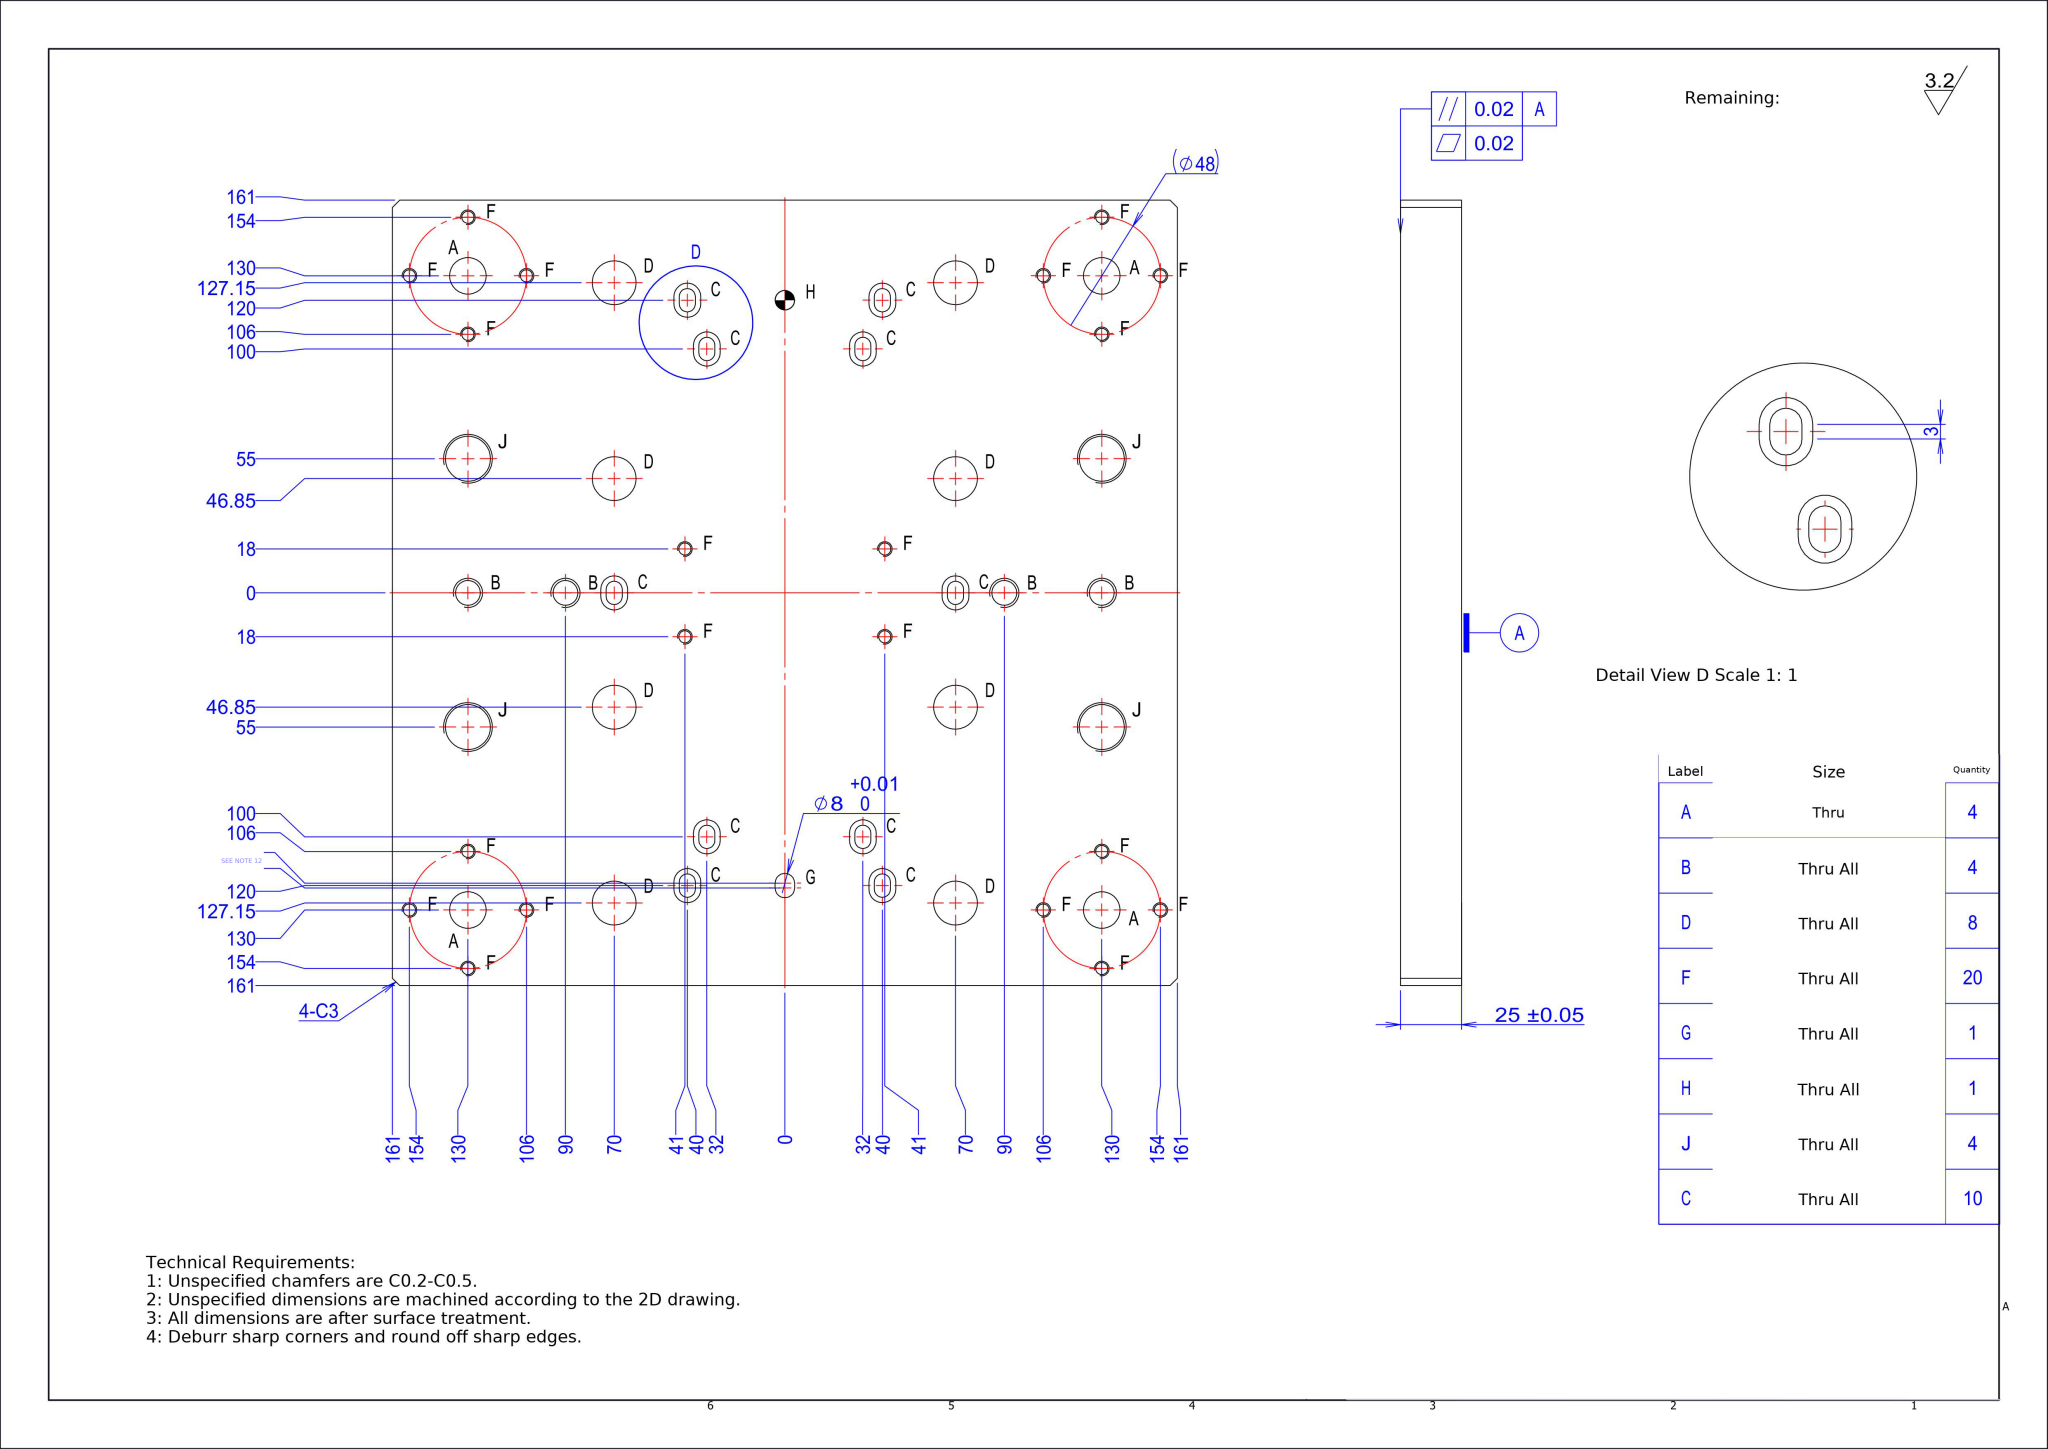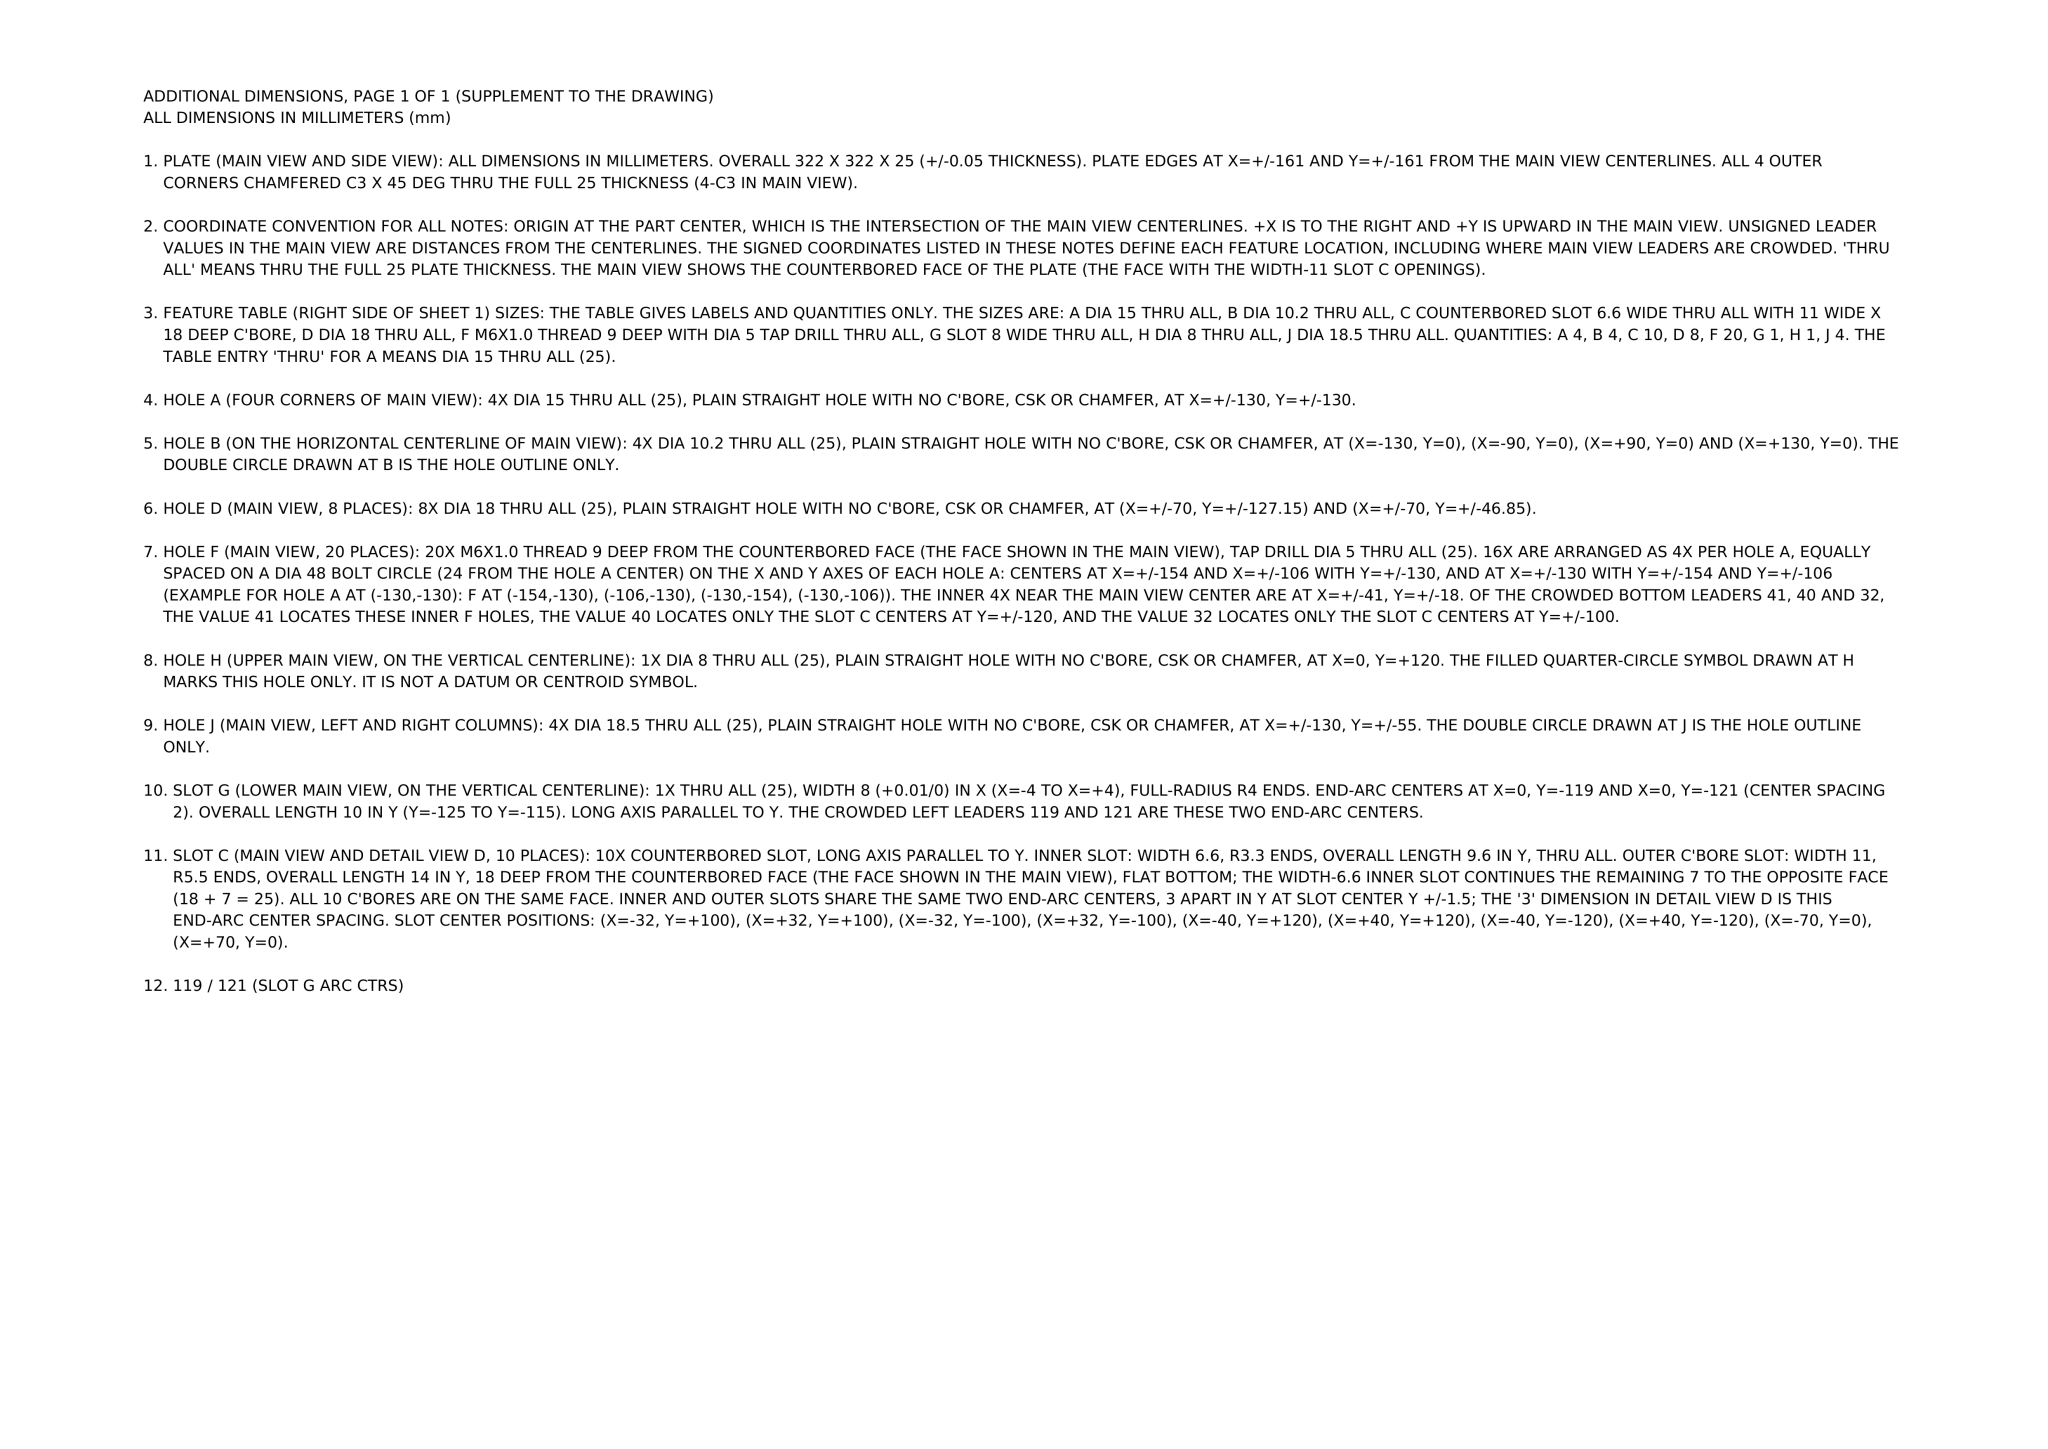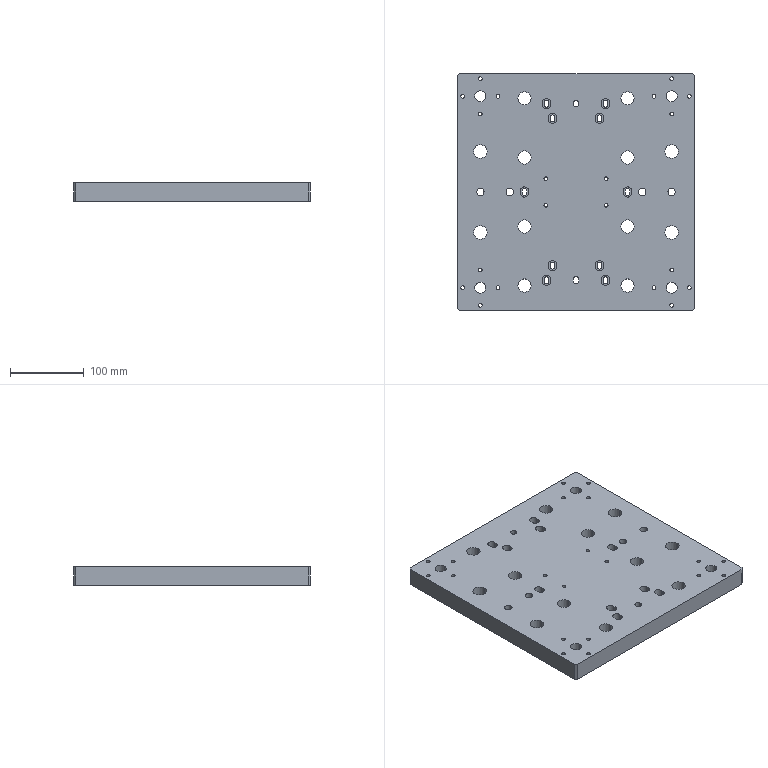Part | NX | mm | 1 solid | 186 faces | box 322 x 322 x 25 mm | volume 2448476 mm3 | cylinder 124 | plane 62 | commonest cylinder face diameters 5 x40 6.6 x20 11 x20 18 x16 10.2 x8 18.5 x8 15 x8 8 x4